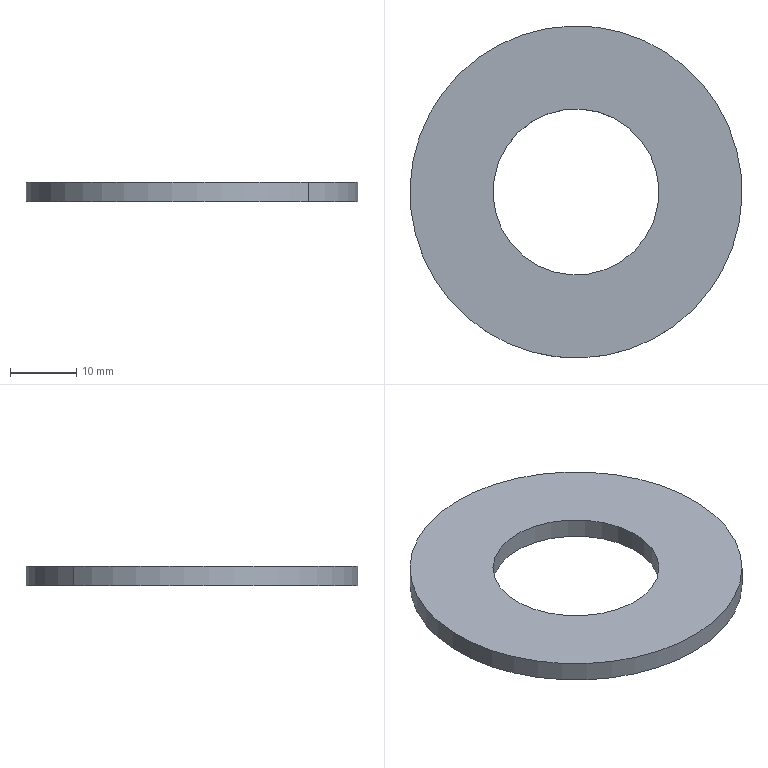Component | SolidWorks | 3Gasket0-1 | 1 solid | 6 faces | box 50 x 50 x 3 mm | volume 4418 mm3 | cylinder 4 | plane 2 | commonest cylinder face diameters 25 x2 50 x2
build123d program:
from build123d import *

# Parameters (mm, degrees)
SKETCH1_R           = 25
SKETCH1_R_2         = 12.5
BOSS_EXTRUDE1_DEPTH = 3


with BuildPart() as part:
    # Sketch1 → Boss-Extrude1 (new body)
    with BuildSketch(Plane.XY):
        Circle(SKETCH1_R)
        Circle(SKETCH1_R_2, mode=Mode.SUBTRACT)
    extrude(amount=BOSS_EXTRUDE1_DEPTH)


solid = part.part

# Placed as in the assembly
solid = solid.moved(Location((-15.093, -37.782, 215.255), (0, 0, 0)))
STEP:
#1=COLOUR_RGB('',0.7922,0.8196,0.9333);
#2=FILL_AREA_STYLE_COLOUR('',#1);
#3=FILL_AREA_STYLE('',(#2));
#4=SURFACE_STYLE_FILL_AREA(#3);
#5=SURFACE_SIDE_STYLE('',(#4));
#6=SURFACE_STYLE_USAGE(.BOTH.,#5);
#7=PRESENTATION_STYLE_ASSIGNMENT((#6));
#8=CARTESIAN_POINT('',(-0.9392,-1.137,8.593));
#9=VERTEX_POINT('',#8);
#10=CARTESIAN_POINT('',(-0.2492,-1.838,8.593));
#11=VERTEX_POINT('',#10);
#12=CARTESIAN_POINT('',(-0.5942,-1.487,8.593));
#13=DIRECTION('',(0.,0.,1.));
#14=DIRECTION('',(0.701,-0.7131,0.));
#15=AXIS2_PLACEMENT_3D('',#12,#13,#14);
#16=CIRCLE('',#15,0.4921);
#17=EDGE_CURVE('',#9,#11,#16,.T.);
#18=ORIENTED_EDGE('',*,*,#17,.T.);
#19=CARTESIAN_POINT('',(-0.2492,-1.838,8.475));
#20=VERTEX_POINT('',#19);
#21=CARTESIAN_POINT('',(-0.2492,-1.838,8.593));
#22=DIRECTION('',(0.,0.,-1.));
#23=VECTOR('',#22,39.37);
#24=LINE('',#21,#23);
#25=EDGE_CURVE('',#11,#20,#24,.T.);
#26=ORIENTED_EDGE('',*,*,#25,.T.);
#27=CARTESIAN_POINT('',(-0.9392,-1.137,8.475));
#28=VERTEX_POINT('',#27);
#29=CARTESIAN_POINT('',(-0.5942,-1.487,8.475));
#30=DIRECTION('',(0.,0.,1.));
#31=DIRECTION('',(0.701,-0.7131,0.));
#32=AXIS2_PLACEMENT_3D('',#29,#30,#31);
#33=CIRCLE('',#32,0.4921);
#34=EDGE_CURVE('',#28,#20,#33,.T.);
#35=ORIENTED_EDGE('',*,*,#34,.F.);
#36=CARTESIAN_POINT('',(-0.9392,-1.137,8.593));
#37=DIRECTION('',(0.,0.,-1.));
#38=VECTOR('',#37,39.37);
#39=LINE('',#36,#38);
#40=EDGE_CURVE('',#9,#28,#39,.T.);
#41=ORIENTED_EDGE('',*,*,#40,.F.);
#42=EDGE_LOOP('',(#18,#26,#35,#41));
#43=FACE_OUTER_BOUND('',#42,.T.);
#44=CARTESIAN_POINT('',(-0.5942,-1.487,8.593));
#45=DIRECTION('',(0.,0.,-1.));
#46=DIRECTION('',(-0.701,0.7131,0.));
#47=AXIS2_PLACEMENT_3D('',#44,#45,#46);
#48=CYLINDRICAL_SURFACE('',#47,0.4921);
#49=ADVANCED_FACE('',(#43),#48,.F.);
#50=CARTESIAN_POINT('',(0.09575,-2.189,8.593));
#51=VERTEX_POINT('',#50);
#52=CARTESIAN_POINT('',(-1.284,-0.7855,8.593));
#53=VERTEX_POINT('',#52);
#54=CARTESIAN_POINT('',(-0.5942,-1.487,8.593));
#55=DIRECTION('',(0.,0.,1.));
#56=DIRECTION('',(0.701,-0.7131,0.));
#57=AXIS2_PLACEMENT_3D('',#54,#55,#56);
#58=CIRCLE('',#57,0.9843);
#59=EDGE_CURVE('',#51,#53,#58,.T.);
#60=ORIENTED_EDGE('',*,*,#59,.F.);
#61=CARTESIAN_POINT('',(0.09575,-2.189,8.475));
#62=VERTEX_POINT('',#61);
#63=CARTESIAN_POINT('',(0.09575,-2.189,8.593));
#64=DIRECTION('',(0.,0.,-1.));
#65=VECTOR('',#64,39.37);
#66=LINE('',#63,#65);
#67=EDGE_CURVE('',#51,#62,#66,.T.);
#68=ORIENTED_EDGE('',*,*,#67,.T.);
#69=CARTESIAN_POINT('',(-1.284,-0.7855,8.475));
#70=VERTEX_POINT('',#69);
#71=CARTESIAN_POINT('',(-0.5942,-1.487,8.475));
#72=DIRECTION('',(0.,0.,1.));
#73=DIRECTION('',(0.701,-0.7131,0.));
#74=AXIS2_PLACEMENT_3D('',#71,#72,#73);
#75=CIRCLE('',#74,0.9843);
#76=EDGE_CURVE('',#62,#70,#75,.T.);
#77=ORIENTED_EDGE('',*,*,#76,.T.);
#78=CARTESIAN_POINT('',(-1.284,-0.7855,8.593));
#79=DIRECTION('',(0.,0.,-1.));
#80=VECTOR('',#79,39.37);
#81=LINE('',#78,#80);
#82=EDGE_CURVE('',#53,#70,#81,.T.);
#83=ORIENTED_EDGE('',*,*,#82,.F.);
#84=EDGE_LOOP('',(#60,#68,#77,#83));
#85=FACE_OUTER_BOUND('',#84,.T.);
#86=CARTESIAN_POINT('',(-0.5942,-1.487,8.593));
#87=DIRECTION('',(0.,0.,-1.));
#88=DIRECTION('',(-0.701,0.7131,0.));
#89=AXIS2_PLACEMENT_3D('',#86,#87,#88);
#90=CYLINDRICAL_SURFACE('',#89,0.9843);
#91=ADVANCED_FACE('',(#85),#90,.T.);
#92=CARTESIAN_POINT('',(-0.5942,-1.487,8.593));
#93=DIRECTION('',(0.,0.,1.));
#94=DIRECTION('',(0.701,-0.7131,0.));
#95=AXIS2_PLACEMENT_3D('',#92,#93,#94);
#96=CIRCLE('',#95,0.9843);
#97=EDGE_CURVE('',#53,#51,#96,.T.);
#98=ORIENTED_EDGE('',*,*,#97,.T.);
#99=ORIENTED_EDGE('',*,*,#59,.T.);
#100=EDGE_LOOP('',(#98,#99));
#101=FACE_OUTER_BOUND('',#100,.T.);
#102=ORIENTED_EDGE('',*,*,#17,.F.);
#103=CARTESIAN_POINT('',(-0.5942,-1.487,8.593));
#104=DIRECTION('',(0.,0.,1.));
#105=DIRECTION('',(0.701,-0.7131,0.));
#106=AXIS2_PLACEMENT_3D('',#103,#104,#105);
#107=CIRCLE('',#106,0.4921);
#108=EDGE_CURVE('',#11,#9,#107,.T.);
#109=ORIENTED_EDGE('',*,*,#108,.F.);
#110=EDGE_LOOP('',(#102,#109));
#111=FACE_BOUND('',#110,.T.);
#112=CARTESIAN_POINT('',(-0.5942,-1.487,8.593));
#113=DIRECTION('',(0.,0.,1.));
#114=DIRECTION('',(0.701,-0.7131,0.));
#115=AXIS2_PLACEMENT_3D('',#112,#113,#114);
#116=PLANE('',#115);
#117=ADVANCED_FACE('',(#101,#111),#116,.T.);
#118=CARTESIAN_POINT('',(-0.5942,-1.487,8.475));
#119=DIRECTION('',(0.,0.,1.));
#120=DIRECTION('',(0.701,-0.7131,0.));
#121=AXIS2_PLACEMENT_3D('',#118,#119,#120);
#122=CIRCLE('',#121,0.9843);
#123=EDGE_CURVE('',#70,#62,#122,.T.);
#124=ORIENTED_EDGE('',*,*,#123,.F.);
#125=ORIENTED_EDGE('',*,*,#76,.F.);
#126=EDGE_LOOP('',(#124,#125));
#127=FACE_OUTER_BOUND('',#126,.T.);
#128=ORIENTED_EDGE('',*,*,#34,.T.);
#129=CARTESIAN_POINT('',(-0.5942,-1.487,8.475));
#130=DIRECTION('',(0.,0.,1.));
#131=DIRECTION('',(0.701,-0.7131,0.));
#132=AXIS2_PLACEMENT_3D('',#129,#130,#131);
#133=CIRCLE('',#132,0.4921);
#134=EDGE_CURVE('',#20,#28,#133,.T.);
#135=ORIENTED_EDGE('',*,*,#134,.T.);
#136=EDGE_LOOP('',(#128,#135));
#137=FACE_BOUND('',#136,.T.);
#138=CARTESIAN_POINT('',(-0.5942,-1.487,8.475));
#139=DIRECTION('',(0.,0.,1.));
#140=DIRECTION('',(0.701,-0.7131,0.));
#141=AXIS2_PLACEMENT_3D('',#138,#139,#140);
#142=PLANE('',#141);
#143=ADVANCED_FACE('',(#127,#137),#142,.F.);
#144=ORIENTED_EDGE('',*,*,#67,.F.);
#145=ORIENTED_EDGE('',*,*,#97,.F.);
#146=ORIENTED_EDGE('',*,*,#82,.T.);
#147=ORIENTED_EDGE('',*,*,#123,.T.);
#148=EDGE_LOOP('',(#144,#145,#146,#147));
#149=FACE_OUTER_BOUND('',#148,.T.);
#150=CARTESIAN_POINT('',(-0.5942,-1.487,8.593));
#151=DIRECTION('',(0.,0.,-1.));
#152=DIRECTION('',(-0.701,0.7131,0.));
#153=AXIS2_PLACEMENT_3D('',#150,#151,#152);
#154=CYLINDRICAL_SURFACE('',#153,0.9843);
#155=ADVANCED_FACE('',(#149),#154,.T.);
#156=ORIENTED_EDGE('',*,*,#25,.F.);
#157=ORIENTED_EDGE('',*,*,#108,.T.);
#158=ORIENTED_EDGE('',*,*,#40,.T.);
#159=ORIENTED_EDGE('',*,*,#134,.F.);
#160=EDGE_LOOP('',(#156,#157,#158,#159));
#161=FACE_OUTER_BOUND('',#160,.T.);
#162=CARTESIAN_POINT('',(-0.5942,-1.487,8.593));
#163=DIRECTION('',(0.,0.,-1.));
#164=DIRECTION('',(-0.701,0.7131,0.));
#165=AXIS2_PLACEMENT_3D('',#162,#163,#164);
#166=CYLINDRICAL_SURFACE('',#165,0.4921);
#167=ADVANCED_FACE('',(#161),#166,.F.);
#168=CLOSED_SHELL('',(#49,#91,#117,#143,#155,#167));
#169=MANIFOLD_SOLID_BREP('',#168);
#170=STYLED_ITEM('',(#7),#169);
#171=PRESENTATION_LAYER_ASSIGNMENT('','',(#170));
#172=(LENGTH_UNIT()NAMED_UNIT(*)SI_UNIT($,.METRE.));
#173=LENGTH_MEASURE_WITH_UNIT(LENGTH_MEASURE(0.0254),#172);
#174=DIMENSIONAL_EXPONENTS(1.,0.,0.,0.,0.,0.,0.);
#175=(CONVERSION_BASED_UNIT('',#173)LENGTH_UNIT()NAMED_UNIT(#174));
#176=UNCERTAINTY_MEASURE_WITH_UNIT(LENGTH_MEASURE(0.00001),#175,'','');
#177=(NAMED_UNIT(*)PLANE_ANGLE_UNIT()SI_UNIT($,.RADIAN.));
#178=(NAMED_UNIT(*)SI_UNIT($,.STERADIAN.)SOLID_ANGLE_UNIT());
#179=(GEOMETRIC_REPRESENTATION_CONTEXT(3)GLOBAL_UNCERTAINTY_ASSIGNED_CONTEXT((#176))GLOBAL_UNIT_ASSIGNED_CONTEXT((#175,#177,#178))REPRESENTATION_CONTEXT('',''));
#180=MECHANICAL_DESIGN_GEOMETRIC_PRESENTATION_REPRESENTATION('',(#170),#179);
#181=CARTESIAN_POINT('',(0.,0.,0.));
#182=DIRECTION('',(0.,0.,1.));
#183=DIRECTION('',(1.,0.,0.));
#184=AXIS2_PLACEMENT_3D('',#181,#182,#183);
#185=(LENGTH_UNIT()NAMED_UNIT(*)SI_UNIT($,.METRE.));
#186=LENGTH_MEASURE_WITH_UNIT(LENGTH_MEASURE(0.0254),#185);
#187=DIMENSIONAL_EXPONENTS(1.,0.,0.,0.,0.,0.,0.);
#188=(CONVERSION_BASED_UNIT('',#186)LENGTH_UNIT()NAMED_UNIT(#187));
#189=UNCERTAINTY_MEASURE_WITH_UNIT(LENGTH_MEASURE(0.00001),#188,'','');
#190=(NAMED_UNIT(*)PLANE_ANGLE_UNIT()SI_UNIT($,.RADIAN.));
#191=(NAMED_UNIT(*)SI_UNIT($,.STERADIAN.)SOLID_ANGLE_UNIT());
#192=(GEOMETRIC_REPRESENTATION_CONTEXT(3)GLOBAL_UNCERTAINTY_ASSIGNED_CONTEXT((#189))GLOBAL_UNIT_ASSIGNED_CONTEXT((#188,#190,#191))REPRESENTATION_CONTEXT('',''));
#193=ADVANCED_BREP_SHAPE_REPRESENTATION('',(#169,#184),#192);